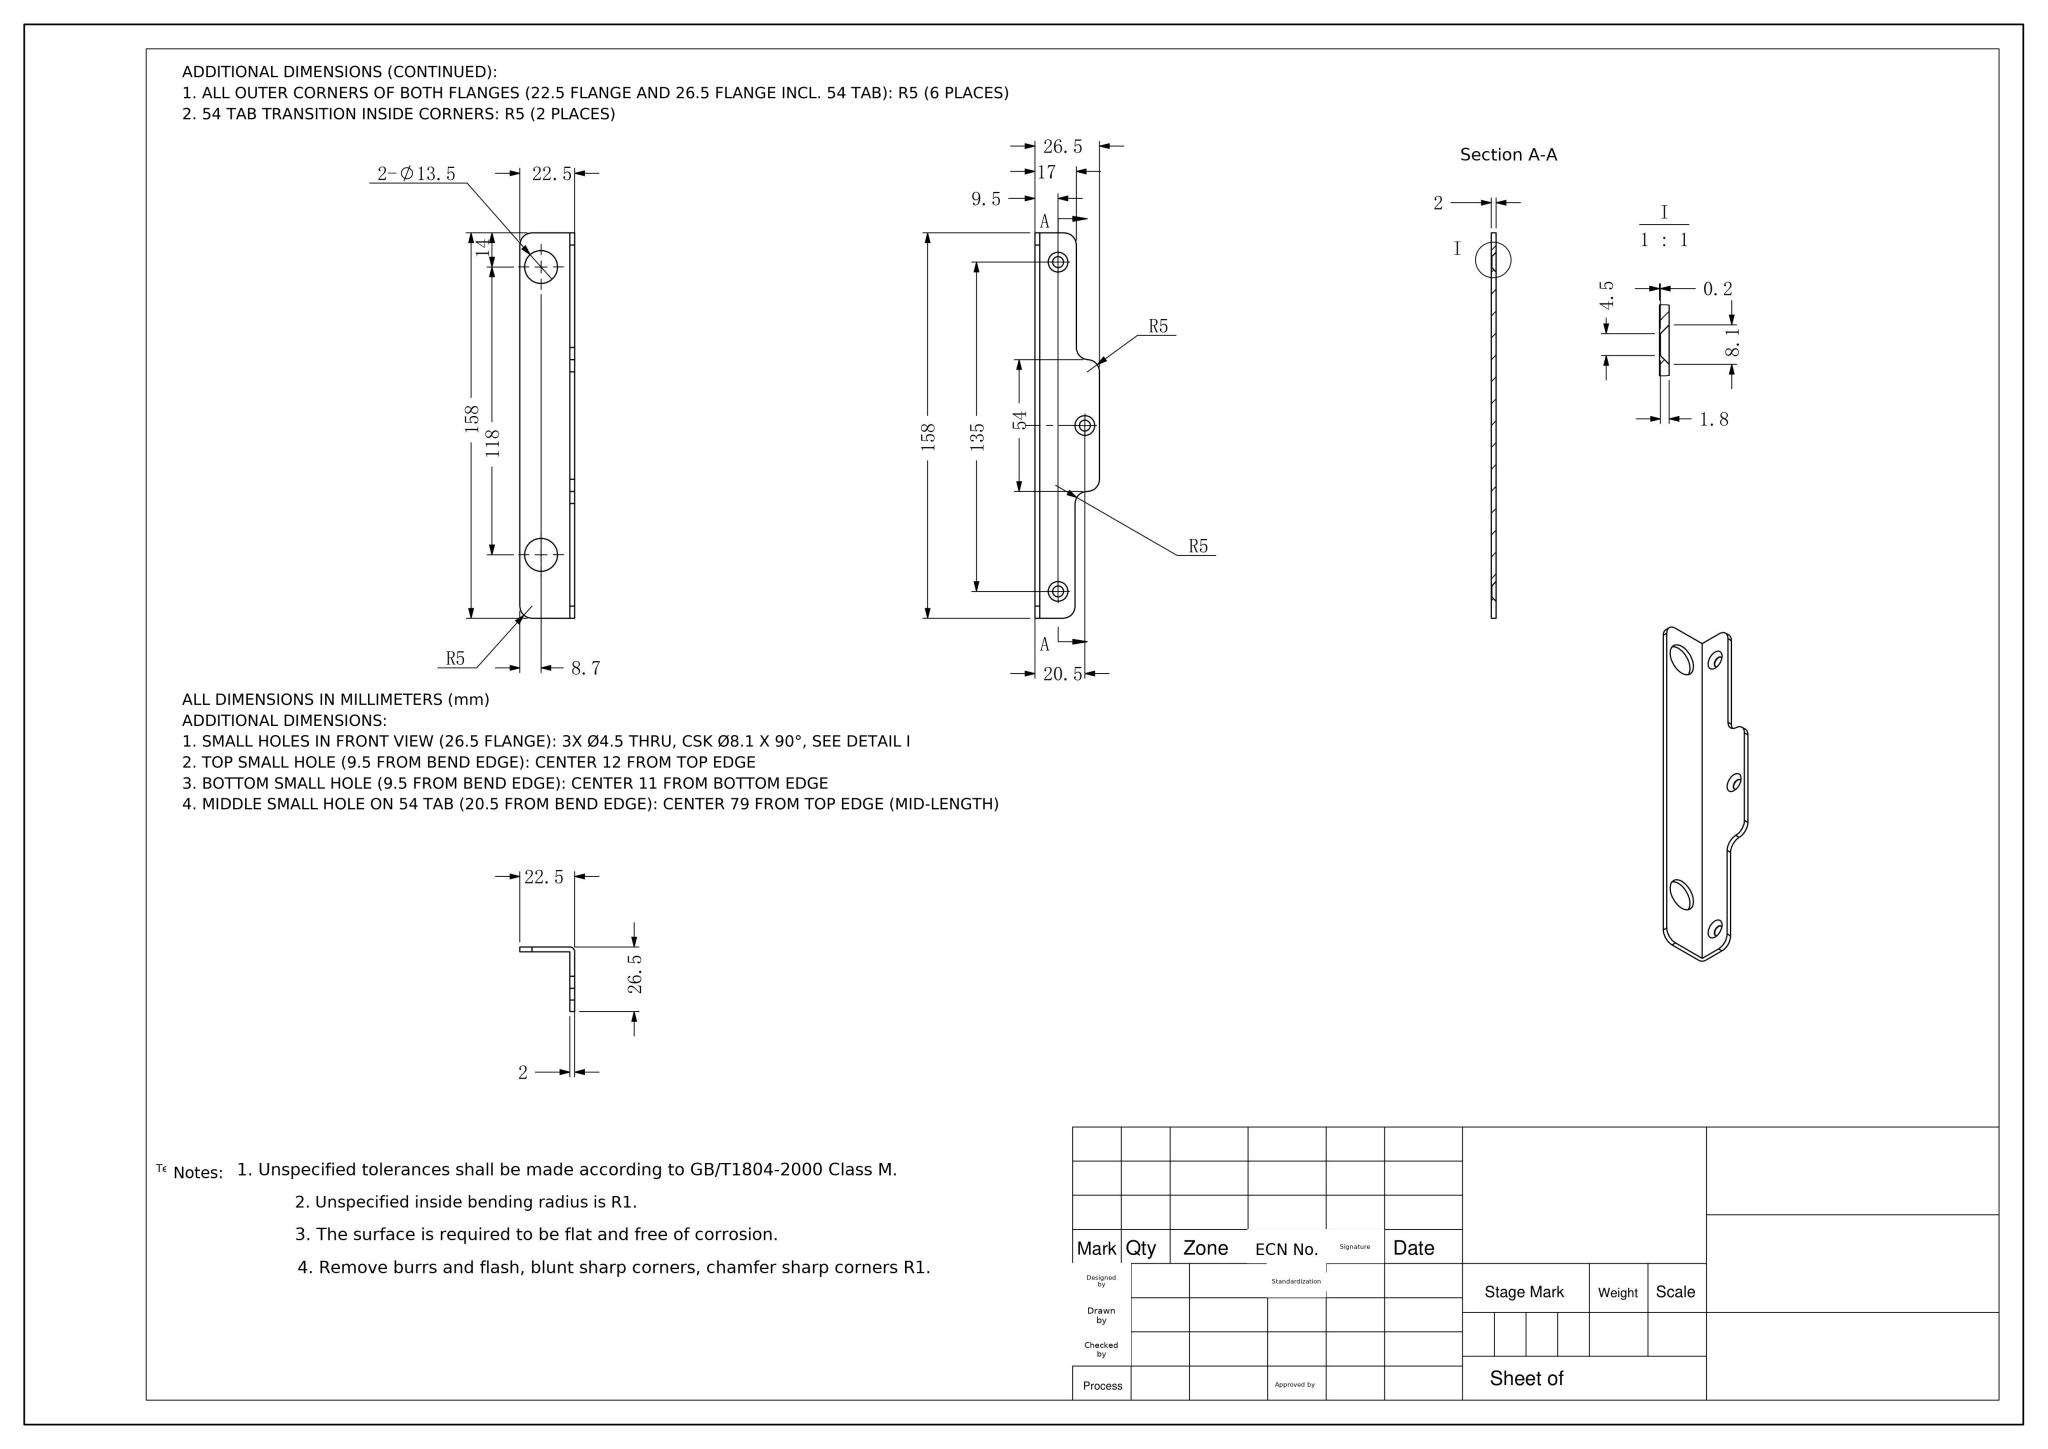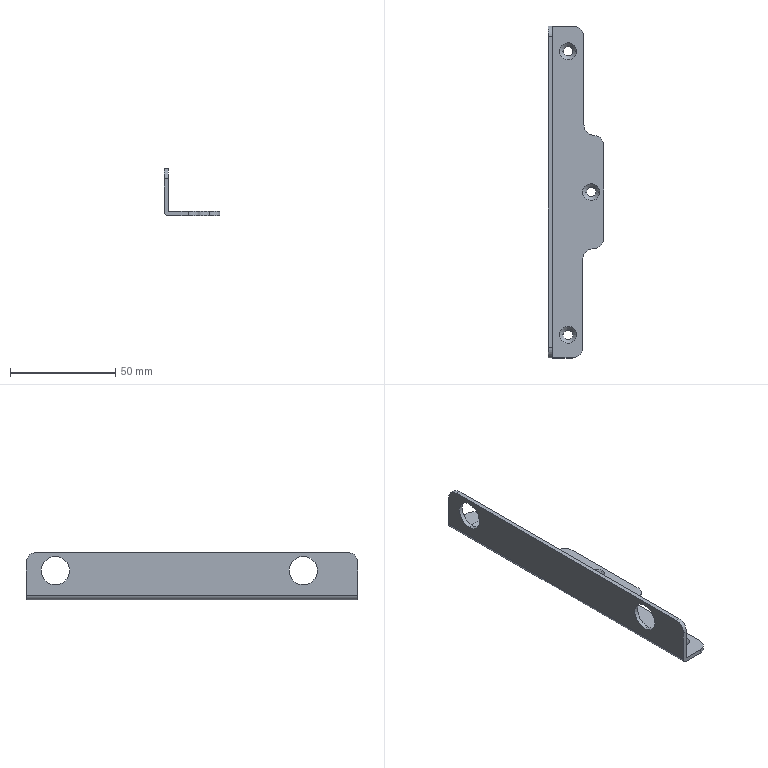Part | NX | mm | 1 solid | 36 faces | box 26.5 x 158 x 22.5 mm | volume 11890 mm3 | cylinder 20 | plane 10 | cone 6 | commonest cylinder face diameters 10 x8 4.5 x6 13.5 x4 0.004 x1 4.004 x1